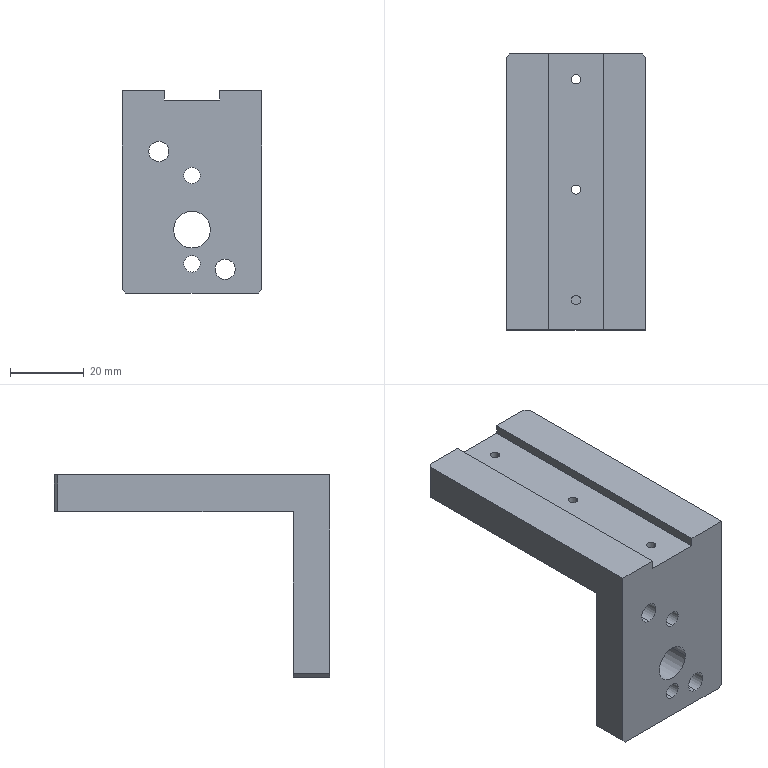Component | SolidWorks | CCDJSGrippingCylinderAngleAluminum01-1 | 1 solid | 33 faces | box 38 x 75 x 55 mm | volume 41060 mm3 | plane 17 | cylinder 16 | commonest cylinder face diameters 2.5 x6 4.5 x4 5.5 x4 10 x2
STEP:
#1=COLOUR_RGB('',0.7922,0.8196,0.9333);
#2=FILL_AREA_STYLE_COLOUR('',#1);
#3=FILL_AREA_STYLE('',(#2));
#4=SURFACE_STYLE_FILL_AREA(#3);
#5=SURFACE_SIDE_STYLE('',(#4));
#6=SURFACE_STYLE_USAGE(.BOTH.,#5);
#7=PRESENTATION_STYLE_ASSIGNMENT((#6));
#8=CARTESIAN_POINT('',(-6.256,14.188,-4.54));
#9=VERTEX_POINT('',#8);
#10=CARTESIAN_POINT('',(-6.256,14.188,-4.363));
#11=VERTEX_POINT('',#10);
#12=CARTESIAN_POINT('',(-6.256,14.188,-4.452));
#13=DIRECTION('',(-0.,1.,0.));
#14=DIRECTION('',(0.,0.,1.));
#15=AXIS2_PLACEMENT_3D('',#12,#13,#14);
#16=CIRCLE('',#15,0.08858);
#17=EDGE_CURVE('',#9,#11,#16,.T.);
#18=ORIENTED_EDGE('',*,*,#17,.F.);
#19=CARTESIAN_POINT('',(-6.256,14.581,-4.54));
#20=VERTEX_POINT('',#19);
#21=CARTESIAN_POINT('',(-6.256,14.188,-4.54));
#22=DIRECTION('',(-0.,1.,0.));
#23=VECTOR('',#22,39.37);
#24=LINE('',#21,#23);
#25=EDGE_CURVE('',#9,#20,#24,.T.);
#26=ORIENTED_EDGE('',*,*,#25,.T.);
#27=CARTESIAN_POINT('',(-6.256,14.581,-4.363));
#28=VERTEX_POINT('',#27);
#29=CARTESIAN_POINT('',(-6.256,14.581,-4.452));
#30=DIRECTION('',(-0.,1.,0.));
#31=DIRECTION('',(0.,0.,1.));
#32=AXIS2_PLACEMENT_3D('',#29,#30,#31);
#33=CIRCLE('',#32,0.08858);
#34=EDGE_CURVE('',#20,#28,#33,.T.);
#35=ORIENTED_EDGE('',*,*,#34,.T.);
#36=CARTESIAN_POINT('',(-6.256,14.188,-4.363));
#37=DIRECTION('',(-0.,1.,0.));
#38=VECTOR('',#37,39.37);
#39=LINE('',#36,#38);
#40=EDGE_CURVE('',#11,#28,#39,.T.);
#41=ORIENTED_EDGE('',*,*,#40,.F.);
#42=EDGE_LOOP('',(#18,#26,#35,#41));
#43=FACE_OUTER_BOUND('',#42,.T.);
#44=CARTESIAN_POINT('',(-6.256,14.188,-4.452));
#45=DIRECTION('',(-0.,1.,0.));
#46=DIRECTION('',(0.,0.,1.));
#47=AXIS2_PLACEMENT_3D('',#44,#45,#46);
#48=CYLINDRICAL_SURFACE('',#47,0.08858);
#49=ADVANCED_FACE('',(#43),#48,.F.);
#50=CARTESIAN_POINT('',(-6.256,14.188,-5.485));
#51=VERTEX_POINT('',#50);
#52=CARTESIAN_POINT('',(-6.256,14.188,-5.308));
#53=VERTEX_POINT('',#52);
#54=CARTESIAN_POINT('',(-6.256,14.188,-5.396));
#55=DIRECTION('',(-0.,1.,0.));
#56=DIRECTION('',(0.,0.,1.));
#57=AXIS2_PLACEMENT_3D('',#54,#55,#56);
#58=CIRCLE('',#57,0.08858);
#59=EDGE_CURVE('',#51,#53,#58,.T.);
#60=ORIENTED_EDGE('',*,*,#59,.F.);
#61=CARTESIAN_POINT('',(-6.256,14.581,-5.485));
#62=VERTEX_POINT('',#61);
#63=CARTESIAN_POINT('',(-6.256,14.188,-5.485));
#64=DIRECTION('',(-0.,1.,0.));
#65=VECTOR('',#64,39.37);
#66=LINE('',#63,#65);
#67=EDGE_CURVE('',#51,#62,#66,.T.);
#68=ORIENTED_EDGE('',*,*,#67,.T.);
#69=CARTESIAN_POINT('',(-6.256,14.581,-5.308));
#70=VERTEX_POINT('',#69);
#71=CARTESIAN_POINT('',(-6.256,14.581,-5.396));
#72=DIRECTION('',(-0.,1.,0.));
#73=DIRECTION('',(0.,0.,1.));
#74=AXIS2_PLACEMENT_3D('',#71,#72,#73);
#75=CIRCLE('',#74,0.08858);
#76=EDGE_CURVE('',#62,#70,#75,.T.);
#77=ORIENTED_EDGE('',*,*,#76,.T.);
#78=CARTESIAN_POINT('',(-6.256,14.188,-5.308));
#79=DIRECTION('',(-0.,1.,0.));
#80=VECTOR('',#79,39.37);
#81=LINE('',#78,#80);
#82=EDGE_CURVE('',#53,#70,#81,.T.);
#83=ORIENTED_EDGE('',*,*,#82,.F.);
#84=EDGE_LOOP('',(#60,#68,#77,#83));
#85=FACE_OUTER_BOUND('',#84,.T.);
#86=CARTESIAN_POINT('',(-6.256,14.188,-5.396));
#87=DIRECTION('',(-0.,1.,0.));
#88=DIRECTION('',(0.,0.,1.));
#89=AXIS2_PLACEMENT_3D('',#86,#87,#88);
#90=CYLINDRICAL_SURFACE('',#89,0.08858);
#91=ADVANCED_FACE('',(#85),#90,.F.);
#92=CARTESIAN_POINT('',(-5.902,14.188,-5.564));
#93=VERTEX_POINT('',#92);
#94=CARTESIAN_POINT('',(-5.902,14.188,-5.347));
#95=VERTEX_POINT('',#94);
#96=CARTESIAN_POINT('',(-5.902,14.188,-5.456));
#97=DIRECTION('',(-0.,1.,0.));
#98=DIRECTION('',(1.,0.,0.));
#99=AXIS2_PLACEMENT_3D('',#96,#97,#98);
#100=CIRCLE('',#99,0.1083);
#101=EDGE_CURVE('',#93,#95,#100,.T.);
#102=ORIENTED_EDGE('',*,*,#101,.F.);
#103=CARTESIAN_POINT('',(-5.902,14.581,-5.564));
#104=VERTEX_POINT('',#103);
#105=CARTESIAN_POINT('',(-5.902,13.755,-5.564));
#106=DIRECTION('',(-0.,1.,0.));
#107=VECTOR('',#106,39.37);
#108=LINE('',#105,#107);
#109=EDGE_CURVE('',#93,#104,#108,.T.);
#110=ORIENTED_EDGE('',*,*,#109,.T.);
#111=CARTESIAN_POINT('',(-5.902,14.581,-5.347));
#112=VERTEX_POINT('',#111);
#113=CARTESIAN_POINT('',(-5.902,14.581,-5.456));
#114=DIRECTION('',(-0.,1.,0.));
#115=DIRECTION('',(0.,0.,1.));
#116=AXIS2_PLACEMENT_3D('',#113,#114,#115);
#117=CIRCLE('',#116,0.1083);
#118=EDGE_CURVE('',#104,#112,#117,.T.);
#119=ORIENTED_EDGE('',*,*,#118,.T.);
#120=CARTESIAN_POINT('',(-5.902,13.755,-5.347));
#121=DIRECTION('',(-0.,1.,0.));
#122=VECTOR('',#121,39.37);
#123=LINE('',#120,#122);
#124=EDGE_CURVE('',#95,#112,#123,.T.);
#125=ORIENTED_EDGE('',*,*,#124,.F.);
#126=EDGE_LOOP('',(#102,#110,#119,#125));
#127=FACE_OUTER_BOUND('',#126,.T.);
#128=CARTESIAN_POINT('',(-5.902,13.755,-5.456));
#129=DIRECTION('',(-0.,1.,0.));
#130=DIRECTION('',(0.,0.,1.));
#131=AXIS2_PLACEMENT_3D('',#128,#129,#130);
#132=CYLINDRICAL_SURFACE('',#131,0.1083);
#133=ADVANCED_FACE('',(#127),#132,.F.);
#134=CARTESIAN_POINT('',(-6.61,14.188,-4.304));
#135=VERTEX_POINT('',#134);
#136=CARTESIAN_POINT('',(-6.61,14.188,-4.087));
#137=VERTEX_POINT('',#136);
#138=CARTESIAN_POINT('',(-6.61,14.188,-4.196));
#139=DIRECTION('',(-0.,1.,0.));
#140=DIRECTION('',(1.,0.,0.));
#141=AXIS2_PLACEMENT_3D('',#138,#139,#140);
#142=CIRCLE('',#141,0.1083);
#143=EDGE_CURVE('',#135,#137,#142,.T.);
#144=ORIENTED_EDGE('',*,*,#143,.F.);
#145=CARTESIAN_POINT('',(-6.61,14.581,-4.304));
#146=VERTEX_POINT('',#145);
#147=CARTESIAN_POINT('',(-6.61,13.755,-4.304));
#148=DIRECTION('',(-0.,1.,0.));
#149=VECTOR('',#148,39.37);
#150=LINE('',#147,#149);
#151=EDGE_CURVE('',#135,#146,#150,.T.);
#152=ORIENTED_EDGE('',*,*,#151,.T.);
#153=CARTESIAN_POINT('',(-6.61,14.581,-4.087));
#154=VERTEX_POINT('',#153);
#155=CARTESIAN_POINT('',(-6.61,14.581,-4.196));
#156=DIRECTION('',(-0.,1.,0.));
#157=DIRECTION('',(0.,0.,1.));
#158=AXIS2_PLACEMENT_3D('',#155,#156,#157);
#159=CIRCLE('',#158,0.1083);
#160=EDGE_CURVE('',#146,#154,#159,.T.);
#161=ORIENTED_EDGE('',*,*,#160,.T.);
#162=CARTESIAN_POINT('',(-6.61,13.755,-4.087));
#163=DIRECTION('',(-0.,1.,0.));
#164=VECTOR('',#163,39.37);
#165=LINE('',#162,#164);
#166=EDGE_CURVE('',#137,#154,#165,.T.);
#167=ORIENTED_EDGE('',*,*,#166,.F.);
#168=EDGE_LOOP('',(#144,#152,#161,#167));
#169=FACE_OUTER_BOUND('',#168,.T.);
#170=CARTESIAN_POINT('',(-6.61,13.755,-4.196));
#171=DIRECTION('',(-0.,1.,0.));
#172=DIRECTION('',(0.,0.,1.));
#173=AXIS2_PLACEMENT_3D('',#170,#171,#172);
#174=CYLINDRICAL_SURFACE('',#173,0.1083);
#175=ADVANCED_FACE('',(#169),#174,.F.);
#176=CARTESIAN_POINT('',(-6.207,14.506,-3.644));
#177=VERTEX_POINT('',#176);
#178=CARTESIAN_POINT('',(-6.305,14.506,-3.644));
#179=VERTEX_POINT('',#178);
#180=CARTESIAN_POINT('',(-6.256,14.506,-3.644));
#181=DIRECTION('',(0.,0.,-1.));
#182=DIRECTION('',(-1.,0.,0.));
#183=AXIS2_PLACEMENT_3D('',#180,#181,#182);
#184=CIRCLE('',#183,0.04921);
#185=EDGE_CURVE('',#177,#179,#184,.T.);
#186=ORIENTED_EDGE('',*,*,#185,.F.);
#187=CARTESIAN_POINT('',(-6.207,14.506,-3.94));
#188=VERTEX_POINT('',#187);
#189=CARTESIAN_POINT('',(-6.207,14.506,-3.94));
#190=DIRECTION('',(0.,0.,-1.));
#191=VECTOR('',#190,39.37);
#192=LINE('',#189,#191);
#193=EDGE_CURVE('',#177,#188,#192,.T.);
#194=ORIENTED_EDGE('',*,*,#193,.T.);
#195=CARTESIAN_POINT('',(-6.305,14.506,-3.94));
#196=VERTEX_POINT('',#195);
#197=CARTESIAN_POINT('',(-6.256,14.506,-3.94));
#198=DIRECTION('',(0.,0.,-1.));
#199=DIRECTION('',(-1.,0.,0.));
#200=AXIS2_PLACEMENT_3D('',#197,#198,#199);
#201=CIRCLE('',#200,0.04921);
#202=EDGE_CURVE('',#188,#196,#201,.T.);
#203=ORIENTED_EDGE('',*,*,#202,.T.);
#204=CARTESIAN_POINT('',(-6.305,14.506,-3.94));
#205=DIRECTION('',(0.,0.,-1.));
#206=VECTOR('',#205,39.37);
#207=LINE('',#204,#206);
#208=EDGE_CURVE('',#179,#196,#207,.T.);
#209=ORIENTED_EDGE('',*,*,#208,.F.);
#210=EDGE_LOOP('',(#186,#194,#203,#209));
#211=FACE_OUTER_BOUND('',#210,.T.);
#212=CARTESIAN_POINT('',(-6.256,14.506,-3.94));
#213=DIRECTION('',(0.,0.,-1.));
#214=DIRECTION('',(-1.,0.,0.));
#215=AXIS2_PLACEMENT_3D('',#212,#213,#214);
#216=CYLINDRICAL_SURFACE('',#215,0.04921);
#217=ADVANCED_FACE('',(#211),#216,.F.);
#218=CARTESIAN_POINT('',(-6.207,15.688,-3.644));
#219=VERTEX_POINT('',#218);
#220=CARTESIAN_POINT('',(-6.305,15.688,-3.644));
#221=VERTEX_POINT('',#220);
#222=CARTESIAN_POINT('',(-6.256,15.688,-3.644));
#223=DIRECTION('',(0.,0.,-1.));
#224=DIRECTION('',(-1.,0.,0.));
#225=AXIS2_PLACEMENT_3D('',#222,#223,#224);
#226=CIRCLE('',#225,0.04921);
#227=EDGE_CURVE('',#219,#221,#226,.T.);
#228=ORIENTED_EDGE('',*,*,#227,.F.);
#229=CARTESIAN_POINT('',(-6.207,15.688,-3.94));
#230=VERTEX_POINT('',#229);
#231=CARTESIAN_POINT('',(-6.207,15.688,-3.94));
#232=DIRECTION('',(0.,0.,-1.));
#233=VECTOR('',#232,39.37);
#234=LINE('',#231,#233);
#235=EDGE_CURVE('',#219,#230,#234,.T.);
#236=ORIENTED_EDGE('',*,*,#235,.T.);
#237=CARTESIAN_POINT('',(-6.305,15.688,-3.94));
#238=VERTEX_POINT('',#237);
#239=CARTESIAN_POINT('',(-6.256,15.688,-3.94));
#240=DIRECTION('',(0.,0.,-1.));
#241=DIRECTION('',(-1.,0.,0.));
#242=AXIS2_PLACEMENT_3D('',#239,#240,#241);
#243=CIRCLE('',#242,0.04921);
#244=EDGE_CURVE('',#230,#238,#243,.T.);
#245=ORIENTED_EDGE('',*,*,#244,.T.);
#246=CARTESIAN_POINT('',(-6.305,15.688,-3.94));
#247=DIRECTION('',(0.,0.,-1.));
#248=VECTOR('',#247,39.37);
#249=LINE('',#246,#248);
#250=EDGE_CURVE('',#221,#238,#249,.T.);
#251=ORIENTED_EDGE('',*,*,#250,.F.);
#252=EDGE_LOOP('',(#228,#236,#245,#251));
#253=FACE_OUTER_BOUND('',#252,.T.);
#254=CARTESIAN_POINT('',(-6.256,15.688,-3.94));
#255=DIRECTION('',(0.,0.,-1.));
#256=DIRECTION('',(-1.,0.,0.));
#257=AXIS2_PLACEMENT_3D('',#254,#255,#256);
#258=CYLINDRICAL_SURFACE('',#257,0.04921);
#259=ADVANCED_FACE('',(#253),#258,.F.);
#260=CARTESIAN_POINT('',(-6.207,16.869,-3.644));
#261=VERTEX_POINT('',#260);
#262=CARTESIAN_POINT('',(-6.305,16.869,-3.644));
#263=VERTEX_POINT('',#262);
#264=CARTESIAN_POINT('',(-6.256,16.869,-3.644));
#265=DIRECTION('',(0.,0.,-1.));
#266=DIRECTION('',(-1.,0.,0.));
#267=AXIS2_PLACEMENT_3D('',#264,#265,#266);
#268=CIRCLE('',#267,0.04921);
#269=EDGE_CURVE('',#261,#263,#268,.T.);
#270=ORIENTED_EDGE('',*,*,#269,.F.);
#271=CARTESIAN_POINT('',(-6.207,16.869,-3.94));
#272=VERTEX_POINT('',#271);
#273=CARTESIAN_POINT('',(-6.207,16.869,-3.94));
#274=DIRECTION('',(0.,0.,-1.));
#275=VECTOR('',#274,39.37);
#276=LINE('',#273,#275);
#277=EDGE_CURVE('',#261,#272,#276,.T.);
#278=ORIENTED_EDGE('',*,*,#277,.T.);
#279=CARTESIAN_POINT('',(-6.305,16.869,-3.94));
#280=VERTEX_POINT('',#279);
#281=CARTESIAN_POINT('',(-6.256,16.869,-3.94));
#282=DIRECTION('',(0.,0.,-1.));
#283=DIRECTION('',(-1.,0.,0.));
#284=AXIS2_PLACEMENT_3D('',#281,#282,#283);
#285=CIRCLE('',#284,0.04921);
#286=EDGE_CURVE('',#272,#280,#285,.T.);
#287=ORIENTED_EDGE('',*,*,#286,.T.);
#288=CARTESIAN_POINT('',(-6.305,16.869,-3.94));
#289=DIRECTION('',(0.,0.,-1.));
#290=VECTOR('',#289,39.37);
#291=LINE('',#288,#290);
#292=EDGE_CURVE('',#263,#280,#291,.T.);
#293=ORIENTED_EDGE('',*,*,#292,.F.);
#294=EDGE_LOOP('',(#270,#278,#287,#293));
#295=FACE_OUTER_BOUND('',#294,.T.);
#296=CARTESIAN_POINT('',(-6.256,16.869,-3.94));
#297=DIRECTION('',(0.,0.,-1.));
#298=DIRECTION('',(-1.,0.,0.));
#299=AXIS2_PLACEMENT_3D('',#296,#297,#298);
#300=CYLINDRICAL_SURFACE('',#299,0.04921);
#301=ADVANCED_FACE('',(#295),#300,.F.);
#302=CARTESIAN_POINT('',(-6.453,14.188,-5.032));
#303=VERTEX_POINT('',#302);
#304=CARTESIAN_POINT('',(-6.059,14.188,-5.032));
#305=VERTEX_POINT('',#304);
#306=CARTESIAN_POINT('',(-6.256,14.188,-5.032));
#307=DIRECTION('',(-0.,1.,0.));
#308=DIRECTION('',(1.,0.,0.));
#309=AXIS2_PLACEMENT_3D('',#306,#307,#308);
#310=CIRCLE('',#309,0.1969);
#311=EDGE_CURVE('',#303,#305,#310,.T.);
#312=ORIENTED_EDGE('',*,*,#311,.F.);
#313=CARTESIAN_POINT('',(-6.453,14.581,-5.032));
#314=VERTEX_POINT('',#313);
#315=CARTESIAN_POINT('',(-6.453,14.581,-5.032));
#316=DIRECTION('',(-0.,1.,0.));
#317=VECTOR('',#316,39.37);
#318=LINE('',#315,#317);
#319=EDGE_CURVE('',#303,#314,#318,.T.);
#320=ORIENTED_EDGE('',*,*,#319,.T.);
#321=CARTESIAN_POINT('',(-6.059,14.581,-5.032));
#322=VERTEX_POINT('',#321);
#323=CARTESIAN_POINT('',(-6.256,14.581,-5.032));
#324=DIRECTION('',(-0.,1.,0.));
#325=DIRECTION('',(1.,0.,0.));
#326=AXIS2_PLACEMENT_3D('',#323,#324,#325);
#327=CIRCLE('',#326,0.1969);
#328=EDGE_CURVE('',#314,#322,#327,.T.);
#329=ORIENTED_EDGE('',*,*,#328,.T.);
#330=CARTESIAN_POINT('',(-6.059,14.581,-5.032));
#331=DIRECTION('',(-0.,1.,0.));
#332=VECTOR('',#331,39.37);
#333=LINE('',#330,#332);
#334=EDGE_CURVE('',#305,#322,#333,.T.);
#335=ORIENTED_EDGE('',*,*,#334,.F.);
#336=EDGE_LOOP('',(#312,#320,#329,#335));
#337=FACE_OUTER_BOUND('',#336,.T.);
#338=CARTESIAN_POINT('',(-6.256,14.581,-5.032));
#339=DIRECTION('',(-0.,1.,0.));
#340=DIRECTION('',(1.,0.,0.));
#341=AXIS2_PLACEMENT_3D('',#338,#339,#340);
#342=CYLINDRICAL_SURFACE('',#341,0.1969);
#343=ADVANCED_FACE('',(#337),#342,.F.);
#344=CARTESIAN_POINT('',(-5.508,17.101,-3.546));
#345=VERTEX_POINT('',#344);
#346=CARTESIAN_POINT('',(-5.508,14.188,-3.546));
#347=VERTEX_POINT('',#346);
#348=CARTESIAN_POINT('',(-5.508,17.14,-3.546));
#349=DIRECTION('',(0.,-1.,-0.));
#350=VECTOR('',#349,39.37);
#351=LINE('',#348,#350);
#352=EDGE_CURVE('',#345,#347,#351,.T.);
#353=ORIENTED_EDGE('',*,*,#352,.F.);
#354=CARTESIAN_POINT('',(-5.547,17.14,-3.546));
#355=VERTEX_POINT('',#354);
#356=CARTESIAN_POINT('',(-5.508,17.101,-3.546));
#357=DIRECTION('',(-0.7071,0.7071,0.));
#358=VECTOR('',#357,39.37);
#359=LINE('',#356,#358);
#360=EDGE_CURVE('',#345,#355,#359,.T.);
#361=ORIENTED_EDGE('',*,*,#360,.T.);
#362=CARTESIAN_POINT('',(-5.959,17.14,-3.546));
#363=VERTEX_POINT('',#362);
#364=CARTESIAN_POINT('',(-5.508,17.14,-3.546));
#365=DIRECTION('',(-1.,-0.,0.));
#366=VECTOR('',#365,39.37);
#367=LINE('',#364,#366);
#368=EDGE_CURVE('',#355,#363,#367,.T.);
#369=ORIENTED_EDGE('',*,*,#368,.T.);
#370=CARTESIAN_POINT('',(-5.959,14.188,-3.546));
#371=VERTEX_POINT('',#370);
#372=CARTESIAN_POINT('',(-5.959,17.14,-3.546));
#373=DIRECTION('',(0.,-1.,-0.));
#374=VECTOR('',#373,39.37);
#375=LINE('',#372,#374);
#376=EDGE_CURVE('',#363,#371,#375,.T.);
#377=ORIENTED_EDGE('',*,*,#376,.T.);
#378=CARTESIAN_POINT('',(-5.508,14.188,-3.546));
#379=DIRECTION('',(-1.,-0.,0.));
#380=VECTOR('',#379,39.37);
#381=LINE('',#378,#380);
#382=EDGE_CURVE('',#347,#371,#381,.T.);
#383=ORIENTED_EDGE('',*,*,#382,.F.);
#384=EDGE_LOOP('',(#353,#361,#369,#377,#383));
#385=FACE_OUTER_BOUND('',#384,.T.);
#386=CARTESIAN_POINT('',(-5.508,17.14,-3.546));
#387=DIRECTION('',(-0.,0.,-1.));
#388=DIRECTION('',(-0.,1.,0.));
#389=AXIS2_PLACEMENT_3D('',#386,#387,#388);
#390=PLANE('',#389);
#391=ADVANCED_FACE('',(#385),#390,.F.);
#392=CARTESIAN_POINT('',(-6.256,14.581,-4.452));
#393=DIRECTION('',(-0.,1.,0.));
#394=DIRECTION('',(0.,0.,1.));
#395=AXIS2_PLACEMENT_3D('',#392,#393,#394);
#396=CIRCLE('',#395,0.08858);
#397=EDGE_CURVE('',#28,#20,#396,.T.);
#398=ORIENTED_EDGE('',*,*,#397,.F.);
#399=ORIENTED_EDGE('',*,*,#34,.F.);
#400=EDGE_LOOP('',(#398,#399));
#401=FACE_BOUND('',#400,.T.);
#402=CARTESIAN_POINT('',(-6.256,14.581,-5.396));
#403=DIRECTION('',(-0.,1.,0.));
#404=DIRECTION('',(0.,0.,1.));
#405=AXIS2_PLACEMENT_3D('',#402,#403,#404);
#406=CIRCLE('',#405,0.08858);
#407=EDGE_CURVE('',#70,#62,#406,.T.);
#408=ORIENTED_EDGE('',*,*,#407,.F.);
#409=ORIENTED_EDGE('',*,*,#76,.F.);
#410=EDGE_LOOP('',(#408,#409));
#411=FACE_BOUND('',#410,.T.);
#412=CARTESIAN_POINT('',(-5.902,14.581,-5.456));
#413=DIRECTION('',(-0.,1.,0.));
#414=DIRECTION('',(0.,0.,1.));
#415=AXIS2_PLACEMENT_3D('',#412,#413,#414);
#416=CIRCLE('',#415,0.1083);
#417=EDGE_CURVE('',#112,#104,#416,.T.);
#418=ORIENTED_EDGE('',*,*,#417,.F.);
#419=ORIENTED_EDGE('',*,*,#118,.F.);
#420=EDGE_LOOP('',(#418,#419));
#421=FACE_BOUND('',#420,.T.);
#422=CARTESIAN_POINT('',(-6.61,14.581,-4.196));
#423=DIRECTION('',(-0.,1.,0.));
#424=DIRECTION('',(0.,0.,1.));
#425=AXIS2_PLACEMENT_3D('',#422,#423,#424);
#426=CIRCLE('',#425,0.1083);
#427=EDGE_CURVE('',#154,#146,#426,.T.);
#428=ORIENTED_EDGE('',*,*,#427,.F.);
#429=ORIENTED_EDGE('',*,*,#160,.F.);
#430=EDGE_LOOP('',(#428,#429));
#431=FACE_BOUND('',#430,.T.);
#432=CARTESIAN_POINT('',(-6.256,14.581,-5.032));
#433=DIRECTION('',(-0.,1.,0.));
#434=DIRECTION('',(1.,0.,0.));
#435=AXIS2_PLACEMENT_3D('',#432,#433,#434);
#436=CIRCLE('',#435,0.1969);
#437=EDGE_CURVE('',#322,#314,#436,.T.);
#438=ORIENTED_EDGE('',*,*,#437,.F.);
#439=ORIENTED_EDGE('',*,*,#328,.F.);
#440=EDGE_LOOP('',(#438,#439));
#441=FACE_BOUND('',#440,.T.);
#442=CARTESIAN_POINT('',(-5.508,14.581,-5.672));
#443=VERTEX_POINT('',#442);
#444=CARTESIAN_POINT('',(-5.508,14.581,-3.94));
#445=VERTEX_POINT('',#444);
#446=CARTESIAN_POINT('',(-5.508,14.581,-5.711));
#447=DIRECTION('',(0.,-0.,1.));
#448=VECTOR('',#447,39.37);
#449=LINE('',#446,#448);
#450=EDGE_CURVE('',#443,#445,#449,.T.);
#451=ORIENTED_EDGE('',*,*,#450,.F.);
#452=CARTESIAN_POINT('',(-5.547,14.581,-5.711));
#453=VERTEX_POINT('',#452);
#454=CARTESIAN_POINT('',(-5.508,14.581,-5.672));
#455=DIRECTION('',(-0.7071,-0.,-0.7071));
#456=VECTOR('',#455,39.37);
#457=LINE('',#454,#456);
#458=EDGE_CURVE('',#443,#453,#457,.T.);
#459=ORIENTED_EDGE('',*,*,#458,.T.);
#460=CARTESIAN_POINT('',(-6.965,14.581,-5.711));
#461=VERTEX_POINT('',#460);
#462=CARTESIAN_POINT('',(-5.508,14.581,-5.711));
#463=DIRECTION('',(-1.,-0.,0.));
#464=VECTOR('',#463,39.37);
#465=LINE('',#462,#464);
#466=EDGE_CURVE('',#453,#461,#465,.T.);
#467=ORIENTED_EDGE('',*,*,#466,.T.);
#468=CARTESIAN_POINT('',(-7.004,14.581,-5.672));
#469=VERTEX_POINT('',#468);
#470=CARTESIAN_POINT('',(-6.965,14.581,-5.711));
#471=DIRECTION('',(-0.7071,-0.,0.7071));
#472=VECTOR('',#471,39.37);
#473=LINE('',#470,#472);
#474=EDGE_CURVE('',#461,#469,#473,.T.);
#475=ORIENTED_EDGE('',*,*,#474,.T.);
#476=CARTESIAN_POINT('',(-7.004,14.581,-3.94));
#477=VERTEX_POINT('',#476);
#478=CARTESIAN_POINT('',(-7.004,14.581,-5.711));
#479=DIRECTION('',(0.,-0.,1.));
#480=VECTOR('',#479,39.37);
#481=LINE('',#478,#480);
#482=EDGE_CURVE('',#469,#477,#481,.T.);
#483=ORIENTED_EDGE('',*,*,#482,.T.);
#484=CARTESIAN_POINT('',(-5.508,14.581,-3.94));
#485=DIRECTION('',(-1.,-0.,0.));
#486=VECTOR('',#485,39.37);
#487=LINE('',#484,#486);
#488=EDGE_CURVE('',#445,#477,#487,.T.);
#489=ORIENTED_EDGE('',*,*,#488,.F.);
#490=EDGE_LOOP('',(#451,#459,#467,#475,#483,#489));
#491=FACE_OUTER_BOUND('',#490,.T.);
#492=CARTESIAN_POINT('',(-5.508,14.581,-5.711));
#493=DIRECTION('',(0.,-1.,-0.));
#494=DIRECTION('',(-0.,0.,-1.));
#495=AXIS2_PLACEMENT_3D('',#492,#493,#494);
#496=PLANE('',#495);
#497=ADVANCED_FACE('',(#401,#411,#421,#431,#441,#491),#496,.F.);
#498=CARTESIAN_POINT('',(-6.256,15.688,-3.94));
#499=DIRECTION('',(0.,0.,-1.));
#500=DIRECTION('',(-1.,0.,0.));
#501=AXIS2_PLACEMENT_3D('',#498,#499,#500);
#502=CIRCLE('',#501,0.04921);
#503=EDGE_CURVE('',#238,#230,#502,.T.);
#504=ORIENTED_EDGE('',*,*,#503,.F.);
#505=ORIENTED_EDGE('',*,*,#244,.F.);
#506=EDGE_LOOP('',(#504,#505));
#507=FACE_BOUND('',#506,.T.);
#508=CARTESIAN_POINT('',(-6.256,16.869,-3.94));
#509=DIRECTION('',(0.,0.,-1.));
#510=DIRECTION('',(-1.,0.,0.));
#511=AXIS2_PLACEMENT_3D('',#508,#509,#510);
#512=CIRCLE('',#511,0.04921);
#513=EDGE_CURVE('',#280,#272,#512,.T.);
#514=ORIENTED_EDGE('',*,*,#513,.F.);
#515=ORIENTED_EDGE('',*,*,#286,.F.);
#516=EDGE_LOOP('',(#514,#515));
#517=FACE_BOUND('',#516,.T.);
#518=CARTESIAN_POINT('',(-7.004,17.101,-3.94));
#519=VERTEX_POINT('',#518);
#520=CARTESIAN_POINT('',(-7.004,14.581,-3.94));
#521=DIRECTION('',(-0.,1.,0.));
#522=VECTOR('',#521,39.37);
#523=LINE('',#520,#522);
#524=EDGE_CURVE('',#477,#519,#523,.T.);
#525=ORIENTED_EDGE('',*,*,#524,.T.);
#526=CARTESIAN_POINT('',(-6.965,17.14,-3.94));
#527=VERTEX_POINT('',#526);
#528=CARTESIAN_POINT('',(-6.965,17.14,-3.94));
#529=DIRECTION('',(0.7071,0.7071,0.));
#530=VECTOR('',#529,39.37);
#531=LINE('',#528,#530);
#532=EDGE_CURVE('',#519,#527,#531,.T.);
#533=ORIENTED_EDGE('',*,*,#532,.T.);
#534=CARTESIAN_POINT('',(-5.547,17.14,-3.94));
#535=VERTEX_POINT('',#534);
#536=CARTESIAN_POINT('',(-5.508,17.14,-3.94));
#537=DIRECTION('',(-1.,-0.,0.));
#538=VECTOR('',#537,39.37);
#539=LINE('',#536,#538);
#540=EDGE_CURVE('',#535,#527,#539,.T.);
#541=ORIENTED_EDGE('',*,*,#540,.F.);
#542=CARTESIAN_POINT('',(-5.508,17.101,-3.94));
#543=VERTEX_POINT('',#542);
#544=CARTESIAN_POINT('',(-5.508,17.101,-3.94));
#545=DIRECTION('',(0.7071,-0.7071,0.));
#546=VECTOR('',#545,39.37);
#547=LINE('',#544,#546);
#548=EDGE_CURVE('',#535,#543,#547,.T.);
#549=ORIENTED_EDGE('',*,*,#548,.T.);
#550=CARTESIAN_POINT('',(-5.508,14.581,-3.94));
#551=DIRECTION('',(-0.,1.,0.));
#552=VECTOR('',#551,39.37);
#553=LINE('',#550,#552);
#554=EDGE_CURVE('',#445,#543,#553,.T.);
#555=ORIENTED_EDGE('',*,*,#554,.F.);
#556=ORIENTED_EDGE('',*,*,#488,.T.);
#557=EDGE_LOOP('',(#525,#533,#541,#549,#555,#556));
#558=FACE_OUTER_BOUND('',#557,.T.);
#559=CARTESIAN_POINT('',(-5.508,14.581,-3.94));
#560=DIRECTION('',(0.,0.,1.));
#561=DIRECTION('',(1.,0.,0.));
#562=AXIS2_PLACEMENT_3D('',#559,#560,#561);
#563=PLANE('',#562);
#564=ADVANCED_FACE('',(#507,#517,#558),#563,.F.);
#565=ORIENTED_EDGE('',*,*,#540,.T.);
#566=CARTESIAN_POINT('',(-6.965,17.14,-3.546));
#567=VERTEX_POINT('',#566);
#568=CARTESIAN_POINT('',(-6.965,17.14,-3.546));
#569=DIRECTION('',(0.,0.,1.));
#570=VECTOR('',#569,39.37);
#571=LINE('',#568,#570);
#572=EDGE_CURVE('',#527,#567,#571,.T.);
#573=ORIENTED_EDGE('',*,*,#572,.T.);
#574=CARTESIAN_POINT('',(-6.553,17.14,-3.546));
#575=VERTEX_POINT('',#574);
#576=CARTESIAN_POINT('',(-5.508,17.14,-3.546));
#577=DIRECTION('',(-1.,-0.,0.));
#578=VECTOR('',#577,39.37);
#579=LINE('',#576,#578);
#580=EDGE_CURVE('',#575,#567,#579,.T.);
#581=ORIENTED_EDGE('',*,*,#580,.F.);
#582=CARTESIAN_POINT('',(-6.553,17.14,-3.644));
#583=VERTEX_POINT('',#582);
#584=CARTESIAN_POINT('',(-6.553,17.14,-3.448));
#585=DIRECTION('',(0.,0.,1.));
#586=VECTOR('',#585,39.37);
#587=LINE('',#584,#586);
#588=EDGE_CURVE('',#583,#575,#587,.T.);
#589=ORIENTED_EDGE('',*,*,#588,.F.);
#590=CARTESIAN_POINT('',(-5.959,17.14,-3.644));
#591=VERTEX_POINT('',#590);
#592=CARTESIAN_POINT('',(-5.959,17.14,-3.644));
#593=DIRECTION('',(-1.,-0.,0.));
#594=VECTOR('',#593,39.37);
#595=LINE('',#592,#594);
#596=EDGE_CURVE('',#591,#583,#595,.T.);
#597=ORIENTED_EDGE('',*,*,#596,.F.);
#598=CARTESIAN_POINT('',(-5.959,17.14,-3.448));
#599=DIRECTION('',(0.,0.,-1.));
#600=VECTOR('',#599,39.37);
#601=LINE('',#598,#600);
#602=EDGE_CURVE('',#363,#591,#601,.T.);
#603=ORIENTED_EDGE('',*,*,#602,.F.);
#604=ORIENTED_EDGE('',*,*,#368,.F.);
#605=CARTESIAN_POINT('',(-5.547,17.14,-3.94));
#606=DIRECTION('',(0.,0.,-1.));
#607=VECTOR('',#606,39.37);
#608=LINE('',#605,#607);
#609=EDGE_CURVE('',#355,#535,#608,.T.);
#610=ORIENTED_EDGE('',*,*,#609,.T.);
#611=EDGE_LOOP('',(#565,#573,#581,#589,#597,#603,#604,#610));
#612=FACE_OUTER_BOUND('',#611,.T.);
#613=CARTESIAN_POINT('',(-5.508,17.14,-3.94));
#614=DIRECTION('',(0.,-1.,0.));
#615=DIRECTION('',(-1.,-0.,0.));
#616=AXIS2_PLACEMENT_3D('',#613,#614,#615);
#617=PLANE('',#616);
#618=ADVANCED_FACE('',(#612),#617,.F.);
#619=ORIENTED_EDGE('',*,*,#580,.T.);
#620=CARTESIAN_POINT('',(-7.004,17.101,-3.546));
#621=VERTEX_POINT('',#620);
#622=CARTESIAN_POINT('',(-6.965,17.14,-3.546));
#623=DIRECTION('',(-0.7071,-0.7071,-0.));
#624=VECTOR('',#623,39.37);
#625=LINE('',#622,#624);
#626=EDGE_CURVE('',#567,#621,#625,.T.);
#627=ORIENTED_EDGE('',*,*,#626,.T.);
#628=CARTESIAN_POINT('',(-7.004,14.188,-3.546));
#629=VERTEX_POINT('',#628);
#630=CARTESIAN_POINT('',(-7.004,17.14,-3.546));
#631=DIRECTION('',(0.,-1.,-0.));
#632=VECTOR('',#631,39.37);
#633=LINE('',#630,#632);
#634=EDGE_CURVE('',#621,#629,#633,.T.);
#635=ORIENTED_EDGE('',*,*,#634,.T.);
#636=CARTESIAN_POINT('',(-6.553,14.188,-3.546));
#637=VERTEX_POINT('',#636);
#638=CARTESIAN_POINT('',(-5.508,14.188,-3.546));
#639=DIRECTION('',(-1.,-0.,0.));
#640=VECTOR('',#639,39.37);
#641=LINE('',#638,#640);
#642=EDGE_CURVE('',#637,#629,#641,.T.);
#643=ORIENTED_EDGE('',*,*,#642,.F.);
#644=CARTESIAN_POINT('',(-6.553,17.14,-3.546));
#645=DIRECTION('',(-0.,1.,0.));
#646=VECTOR('',#645,39.37);
#647=LINE('',#644,#646);
#648=EDGE_CURVE('',#637,#575,#647,.T.);
#649=ORIENTED_EDGE('',*,*,#648,.T.);
#650=EDGE_LOOP('',(#619,#627,#635,#643,#649));
#651=FACE_OUTER_BOUND('',#650,.T.);
#652=CARTESIAN_POINT('',(-5.508,17.14,-3.546));
#653=DIRECTION('',(-0.,0.,-1.));
#654=DIRECTION('',(-0.,1.,0.));
#655=AXIS2_PLACEMENT_3D('',#652,#653,#654);
#656=PLANE('',#655);
#657=ADVANCED_FACE('',(#651),#656,.F.);
#658=CARTESIAN_POINT('',(-6.256,14.188,-4.452));
#659=DIRECTION('',(-0.,1.,0.));
#660=DIRECTION('',(0.,0.,1.));
#661=AXIS2_PLACEMENT_3D('',#658,#659,#660);
#662=CIRCLE('',#661,0.08858);
#663=EDGE_CURVE('',#11,#9,#662,.T.);
#664=ORIENTED_EDGE('',*,*,#663,.T.);
#665=ORIENTED_EDGE('',*,*,#17,.T.);
#666=EDGE_LOOP('',(#664,#665));
#667=FACE_BOUND('',#666,.T.);
#668=CARTESIAN_POINT('',(-6.256,14.188,-5.396));
#669=DIRECTION('',(-0.,1.,0.));
#670=DIRECTION('',(0.,0.,1.));
#671=AXIS2_PLACEMENT_3D('',#668,#669,#670);
#672=CIRCLE('',#671,0.08858);
#673=EDGE_CURVE('',#53,#51,#672,.T.);
#674=ORIENTED_EDGE('',*,*,#673,.T.);
#675=ORIENTED_EDGE('',*,*,#59,.T.);
#676=EDGE_LOOP('',(#674,#675));
#677=FACE_BOUND('',#676,.T.);
#678=CARTESIAN_POINT('',(-5.902,14.188,-5.456));
#679=DIRECTION('',(-0.,1.,0.));
#680=DIRECTION('',(1.,0.,0.));
#681=AXIS2_PLACEMENT_3D('',#678,#679,#680);
#682=CIRCLE('',#681,0.1083);
#683=EDGE_CURVE('',#95,#93,#682,.T.);
#684=ORIENTED_EDGE('',*,*,#683,.T.);
#685=ORIENTED_EDGE('',*,*,#101,.T.);
#686=EDGE_LOOP('',(#684,#685));
#687=FACE_BOUND('',#686,.T.);
#688=CARTESIAN_POINT('',(-6.61,14.188,-4.196));
#689=DIRECTION('',(-0.,1.,0.));
#690=DIRECTION('',(1.,0.,0.));
#691=AXIS2_PLACEMENT_3D('',#688,#689,#690);
#692=CIRCLE('',#691,0.1083);
#693=EDGE_CURVE('',#137,#135,#692,.T.);
#694=ORIENTED_EDGE('',*,*,#693,.T.);
#695=ORIENTED_EDGE('',*,*,#143,.T.);
#696=EDGE_LOOP('',(#694,#695));
#697=FACE_BOUND('',#696,.T.);
#698=CARTESIAN_POINT('',(-6.256,14.188,-5.032));
#699=DIRECTION('',(-0.,1.,0.));
#700=DIRECTION('',(1.,0.,0.));
#701=AXIS2_PLACEMENT_3D('',#698,#699,#700);
#702=CIRCLE('',#701,0.1969);
#703=EDGE_CURVE('',#305,#303,#702,.T.);
#704=ORIENTED_EDGE('',*,*,#703,.T.);
#705=ORIENTED_EDGE('',*,*,#311,.T.);
#706=EDGE_LOOP('',(#704,#705));
#707=FACE_BOUND('',#706,.T.);
#708=CARTESIAN_POINT('',(-5.547,14.188,-5.711));
#709=VERTEX_POINT('',#708);
#710=CARTESIAN_POINT('',(-6.965,14.188,-5.711));
#711=VERTEX_POINT('',#710);
#712=CARTESIAN_POINT('',(-5.508,14.188,-5.711));
#713=DIRECTION('',(-1.,-0.,0.));
#714=VECTOR('',#713,39.37);
#715=LINE('',#712,#714);
#716=EDGE_CURVE('',#709,#711,#715,.T.);
#717=ORIENTED_EDGE('',*,*,#716,.F.);
#718=CARTESIAN_POINT('',(-5.508,14.188,-5.672));
#719=VERTEX_POINT('',#718);
#720=CARTESIAN_POINT('',(-5.508,14.188,-5.672));
#721=DIRECTION('',(0.7071,0.,0.7071));
#722=VECTOR('',#721,39.37);
#723=LINE('',#720,#722);
#724=EDGE_CURVE('',#709,#719,#723,.T.);
#725=ORIENTED_EDGE('',*,*,#724,.T.);
#726=CARTESIAN_POINT('',(-5.508,14.188,-3.546));
#727=DIRECTION('',(0.,0.,-1.));
#728=VECTOR('',#727,39.37);
#729=LINE('',#726,#728);
#730=EDGE_CURVE('',#347,#719,#729,.T.);
#731=ORIENTED_EDGE('',*,*,#730,.F.);
#732=ORIENTED_EDGE('',*,*,#382,.T.);
#733=CARTESIAN_POINT('',(-5.959,14.188,-3.644));
#734=VERTEX_POINT('',#733);
#735=CARTESIAN_POINT('',(-5.959,14.188,-3.546));
#736=DIRECTION('',(0.,0.,-1.));
#737=VECTOR('',#736,39.37);
#738=LINE('',#735,#737);
#739=EDGE_CURVE('',#371,#734,#738,.T.);
#740=ORIENTED_EDGE('',*,*,#739,.T.);
#741=CARTESIAN_POINT('',(-6.553,14.188,-3.644));
#742=VERTEX_POINT('',#741);
#743=CARTESIAN_POINT('',(-5.508,14.188,-3.644));
#744=DIRECTION('',(-1.,-0.,0.));
#745=VECTOR('',#744,39.37);
#746=LINE('',#743,#745);
#747=EDGE_CURVE('',#734,#742,#746,.T.);
#748=ORIENTED_EDGE('',*,*,#747,.T.);
#749=CARTESIAN_POINT('',(-6.553,14.188,-3.546));
#750=DIRECTION('',(0.,0.,1.));
#751=VECTOR('',#750,39.37);
#752=LINE('',#749,#751);
#753=EDGE_CURVE('',#742,#637,#752,.T.);
#754=ORIENTED_EDGE('',*,*,#753,.T.);
#755=ORIENTED_EDGE('',*,*,#642,.T.);
#756=CARTESIAN_POINT('',(-7.004,14.188,-5.672));
#757=VERTEX_POINT('',#756);
#758=CARTESIAN_POINT('',(-7.004,14.188,-3.546));
#759=DIRECTION('',(0.,0.,-1.));
#760=VECTOR('',#759,39.37);
#761=LINE('',#758,#760);
#762=EDGE_CURVE('',#629,#757,#761,.T.);
#763=ORIENTED_EDGE('',*,*,#762,.T.);
#764=CARTESIAN_POINT('',(-6.965,14.188,-5.711));
#765=DIRECTION('',(0.7071,0.,-0.7071));
#766=VECTOR('',#765,39.37);
#767=LINE('',#764,#766);
#768=EDGE_CURVE('',#757,#711,#767,.T.);
#769=ORIENTED_EDGE('',*,*,#768,.T.);
#770=EDGE_LOOP('',(#717,#725,#731,#732,#740,#748,#754,#755,#763,#769));
#771=FACE_OUTER_BOUND('',#770,.T.);
#772=CARTESIAN_POINT('',(-5.508,14.188,-3.546));
#773=DIRECTION('',(-0.,1.,0.));
#774=DIRECTION('',(1.,0.,0.));
#775=AXIS2_PLACEMENT_3D('',#772,#773,#774);
#776=PLANE('',#775);
#777=ADVANCED_FACE('',(#667,#677,#687,#697,#707,#771),#776,.F.);
#778=ORIENTED_EDGE('',*,*,#466,.F.);
#779=CARTESIAN_POINT('',(-5.547,14.188,-5.711));
#780=DIRECTION('',(0.,-1.,0.));
#781=VECTOR('',#780,39.37);
#782=LINE('',#779,#781);
#783=EDGE_CURVE('',#453,#709,#782,.T.);
#784=ORIENTED_EDGE('',*,*,#783,.T.);
#785=ORIENTED_EDGE('',*,*,#716,.T.);
#786=CARTESIAN_POINT('',(-6.965,14.581,-5.711));
#787=DIRECTION('',(-0.,1.,0.));
#788=VECTOR('',#787,39.37);
#789=LINE('',#786,#788);
#790=EDGE_CURVE('',#711,#461,#789,.T.);
#791=ORIENTED_EDGE('',*,*,#790,.T.);
#792=EDGE_LOOP('',(#778,#784,#785,#791));
#793=FACE_OUTER_BOUND('',#792,.T.);
#794=CARTESIAN_POINT('',(-5.508,14.188,-5.711));
#795=DIRECTION('',(0.,0.,1.));
#796=DIRECTION('',(1.,0.,0.));
#797=AXIS2_PLACEMENT_3D('',#794,#795,#796);
#798=PLANE('',#797);
#799=ADVANCED_FACE('',(#793),#798,.F.);
#800=ORIENTED_EDGE('',*,*,#730,.T.);
#801=CARTESIAN_POINT('',(-5.508,14.581,-5.672));
#802=DIRECTION('',(-0.,1.,0.));
#803=VECTOR('',#802,39.37);
#804=LINE('',#801,#803);
#805=EDGE_CURVE('',#719,#443,#804,.T.);
#806=ORIENTED_EDGE('',*,*,#805,.T.);
#807=ORIENTED_EDGE('',*,*,#450,.T.);
#808=ORIENTED_EDGE('',*,*,#554,.T.);
#809=CARTESIAN_POINT('',(-5.508,17.101,-3.94));
#810=DIRECTION('',(0.,0.,1.));
#811=VECTOR('',#810,39.37);
#812=LINE('',#809,#811);
#813=EDGE_CURVE('',#543,#345,#812,.T.);
#814=ORIENTED_EDGE('',*,*,#813,.T.);
#815=ORIENTED_EDGE('',*,*,#352,.T.);
#816=EDGE_LOOP('',(#800,#806,#807,#808,#814,#815));
#817=FACE_OUTER_BOUND('',#816,.T.);
#818=CARTESIAN_POINT('',(-5.508,14.581,-3.94));
#819=DIRECTION('',(-1.,-0.,0.));
#820=DIRECTION('',(0.,0.,1.));
#821=AXIS2_PLACEMENT_3D('',#818,#819,#820);
#822=PLANE('',#821);
#823=ADVANCED_FACE('',(#817),#822,.F.);
#824=ORIENTED_EDGE('',*,*,#482,.F.);
#825=CARTESIAN_POINT('',(-7.004,14.188,-5.672));
#826=DIRECTION('',(0.,-1.,0.));
#827=VECTOR('',#826,39.37);
#828=LINE('',#825,#827);
#829=EDGE_CURVE('',#469,#757,#828,.T.);
#830=ORIENTED_EDGE('',*,*,#829,.T.);
#831=ORIENTED_EDGE('',*,*,#762,.F.);
#832=ORIENTED_EDGE('',*,*,#634,.F.);
#833=CARTESIAN_POINT('',(-7.004,17.101,-3.94));
#834=DIRECTION('',(0.,0.,-1.));
#835=VECTOR('',#834,39.37);
#836=LINE('',#833,#835);
#837=EDGE_CURVE('',#621,#519,#836,.T.);
#838=ORIENTED_EDGE('',*,*,#837,.T.);
#839=ORIENTED_EDGE('',*,*,#524,.F.);
#840=EDGE_LOOP('',(#824,#830,#831,#832,#838,#839));
#841=FACE_OUTER_BOUND('',#840,.T.);
#842=CARTESIAN_POINT('',(-7.004,14.581,-3.94));
#843=DIRECTION('',(-1.,-0.,0.));
#844=DIRECTION('',(0.,0.,1.));
#845=AXIS2_PLACEMENT_3D('',#842,#843,#844);
#846=PLANE('',#845);
#847=ADVANCED_FACE('',(#841),#846,.T.);
#848=CARTESIAN_POINT('',(-6.256,14.506,-3.644));
#849=DIRECTION('',(0.,0.,-1.));
#850=DIRECTION('',(-1.,0.,0.));
#851=AXIS2_PLACEMENT_3D('',#848,#849,#850);
#852=CIRCLE('',#851,0.04921);
#853=EDGE_CURVE('',#179,#177,#852,.T.);
#854=ORIENTED_EDGE('',*,*,#853,.T.);
#855=ORIENTED_EDGE('',*,*,#185,.T.);
#856=EDGE_LOOP('',(#854,#855));
#857=FACE_BOUND('',#856,.T.);
#858=CARTESIAN_POINT('',(-6.256,15.688,-3.644));
#859=DIRECTION('',(0.,0.,-1.));
#860=DIRECTION('',(-1.,0.,0.));
#861=AXIS2_PLACEMENT_3D('',#858,#859,#860);
#862=CIRCLE('',#861,0.04921);
#863=EDGE_CURVE('',#221,#219,#862,.T.);
#864=ORIENTED_EDGE('',*,*,#863,.T.);
#865=ORIENTED_EDGE('',*,*,#227,.T.);
#866=EDGE_LOOP('',(#864,#865));
#867=FACE_BOUND('',#866,.T.);
#868=CARTESIAN_POINT('',(-6.256,16.869,-3.644));
#869=DIRECTION('',(0.,0.,-1.));
#870=DIRECTION('',(-1.,0.,0.));
#871=AXIS2_PLACEMENT_3D('',#868,#869,#870);
#872=CIRCLE('',#871,0.04921);
#873=EDGE_CURVE('',#263,#261,#872,.T.);
#874=ORIENTED_EDGE('',*,*,#873,.T.);
#875=ORIENTED_EDGE('',*,*,#269,.T.);
#876=EDGE_LOOP('',(#874,#875));
#877=FACE_BOUND('',#876,.T.);
#878=CARTESIAN_POINT('',(-5.959,12.652,-3.644));
#879=DIRECTION('',(-0.,1.,0.));
#880=VECTOR('',#879,39.37);
#881=LINE('',#878,#880);
#882=EDGE_CURVE('',#734,#591,#881,.T.);
#883=ORIENTED_EDGE('',*,*,#882,.T.);
#884=ORIENTED_EDGE('',*,*,#596,.T.);
#885=CARTESIAN_POINT('',(-6.553,12.652,-3.644));
#886=DIRECTION('',(-0.,1.,0.));
#887=VECTOR('',#886,39.37);
#888=LINE('',#885,#887);
#889=EDGE_CURVE('',#742,#583,#888,.T.);
#890=ORIENTED_EDGE('',*,*,#889,.F.);
#891=ORIENTED_EDGE('',*,*,#747,.F.);
#892=EDGE_LOOP('',(#883,#884,#890,#891));
#893=FACE_OUTER_BOUND('',#892,.T.);
#894=CARTESIAN_POINT('',(-5.959,12.652,-3.644));
#895=DIRECTION('',(0.,0.,-1.));
#896=DIRECTION('',(-1.,-0.,0.));
#897=AXIS2_PLACEMENT_3D('',#894,#895,#896);
#898=PLANE('',#897);
#899=ADVANCED_FACE('',(#857,#867,#877,#893),#898,.F.);
#900=ORIENTED_EDGE('',*,*,#602,.T.);
#901=ORIENTED_EDGE('',*,*,#882,.F.);
#902=ORIENTED_EDGE('',*,*,#739,.F.);
#903=ORIENTED_EDGE('',*,*,#376,.F.);
#904=EDGE_LOOP('',(#900,#901,#902,#903));
#905=FACE_OUTER_BOUND('',#904,.T.);
#906=CARTESIAN_POINT('',(-5.959,12.652,-3.448));
#907=DIRECTION('',(1.,0.,0.));
#908=DIRECTION('',(0.,0.,-1.));
#909=AXIS2_PLACEMENT_3D('',#906,#907,#908);
#910=PLANE('',#909);
#911=ADVANCED_FACE('',(#905),#910,.F.);
#912=ORIENTED_EDGE('',*,*,#753,.F.);
#913=ORIENTED_EDGE('',*,*,#889,.T.);
#914=ORIENTED_EDGE('',*,*,#588,.T.);
#915=ORIENTED_EDGE('',*,*,#648,.F.);
#916=EDGE_LOOP('',(#912,#913,#914,#915));
#917=FACE_OUTER_BOUND('',#916,.T.);
#918=CARTESIAN_POINT('',(-6.553,12.652,-3.448));
#919=DIRECTION('',(-1.,-0.,0.));
#920=DIRECTION('',(0.,0.,1.));
#921=AXIS2_PLACEMENT_3D('',#918,#919,#920);
#922=PLANE('',#921);
#923=ADVANCED_FACE('',(#917),#922,.F.);
#924=ORIENTED_EDGE('',*,*,#319,.F.);
#925=ORIENTED_EDGE('',*,*,#703,.F.);
#926=ORIENTED_EDGE('',*,*,#334,.T.);
#927=ORIENTED_EDGE('',*,*,#437,.T.);
#928=EDGE_LOOP('',(#924,#925,#926,#927));
#929=FACE_OUTER_BOUND('',#928,.T.);
#930=CARTESIAN_POINT('',(-6.256,14.581,-5.032));
#931=DIRECTION('',(-0.,1.,0.));
#932=DIRECTION('',(1.,0.,0.));
#933=AXIS2_PLACEMENT_3D('',#930,#931,#932);
#934=CYLINDRICAL_SURFACE('',#933,0.1969);
#935=ADVANCED_FACE('',(#929),#934,.F.);
#936=ORIENTED_EDGE('',*,*,#277,.F.);
#937=ORIENTED_EDGE('',*,*,#873,.F.);
#938=ORIENTED_EDGE('',*,*,#292,.T.);
#939=ORIENTED_EDGE('',*,*,#513,.T.);
#940=EDGE_LOOP('',(#936,#937,#938,#939));
#941=FACE_OUTER_BOUND('',#940,.T.);
#942=CARTESIAN_POINT('',(-6.256,16.869,-3.94));
#943=DIRECTION('',(0.,0.,-1.));
#944=DIRECTION('',(-1.,0.,0.));
#945=AXIS2_PLACEMENT_3D('',#942,#943,#944);
#946=CYLINDRICAL_SURFACE('',#945,0.04921);
#947=ADVANCED_FACE('',(#941),#946,.F.);
#948=ORIENTED_EDGE('',*,*,#235,.F.);
#949=ORIENTED_EDGE('',*,*,#863,.F.);
#950=ORIENTED_EDGE('',*,*,#250,.T.);
#951=ORIENTED_EDGE('',*,*,#503,.T.);
#952=EDGE_LOOP('',(#948,#949,#950,#951));
#953=FACE_OUTER_BOUND('',#952,.T.);
#954=CARTESIAN_POINT('',(-6.256,15.688,-3.94));
#955=DIRECTION('',(0.,0.,-1.));
#956=DIRECTION('',(-1.,0.,0.));
#957=AXIS2_PLACEMENT_3D('',#954,#955,#956);
#958=CYLINDRICAL_SURFACE('',#957,0.04921);
#959=ADVANCED_FACE('',(#953),#958,.F.);
#960=CARTESIAN_POINT('',(-6.256,14.506,-3.94));
#961=DIRECTION('',(0.,0.,-1.));
#962=DIRECTION('',(-1.,0.,0.));
#963=AXIS2_PLACEMENT_3D('',#960,#961,#962);
#964=CIRCLE('',#963,0.04921);
#965=EDGE_CURVE('',#196,#188,#964,.T.);
#966=ORIENTED_EDGE('',*,*,#965,.F.);
#967=ORIENTED_EDGE('',*,*,#202,.F.);
#968=EDGE_LOOP('',(#966,#967));
#969=FACE_OUTER_BOUND('',#968,.T.);
#970=CARTESIAN_POINT('',(-6.256,14.556,-3.94));
#971=DIRECTION('',(0.,0.,-1.));
#972=DIRECTION('',(-1.,-0.,0.));
#973=AXIS2_PLACEMENT_3D('',#970,#971,#972);
#974=PLANE('',#973);
#975=ADVANCED_FACE('',(#969),#974,.F.);
#976=ORIENTED_EDGE('',*,*,#193,.F.);
#977=ORIENTED_EDGE('',*,*,#853,.F.);
#978=ORIENTED_EDGE('',*,*,#208,.T.);
#979=ORIENTED_EDGE('',*,*,#965,.T.);
#980=EDGE_LOOP('',(#976,#977,#978,#979));
#981=FACE_OUTER_BOUND('',#980,.T.);
#982=CARTESIAN_POINT('',(-6.256,14.506,-3.94));
#983=DIRECTION('',(0.,0.,-1.));
#984=DIRECTION('',(-1.,0.,0.));
#985=AXIS2_PLACEMENT_3D('',#982,#983,#984);
#986=CYLINDRICAL_SURFACE('',#985,0.04921);
#987=ADVANCED_FACE('',(#981),#986,.F.);
#988=ORIENTED_EDGE('',*,*,#724,.F.);
#989=ORIENTED_EDGE('',*,*,#783,.F.);
#990=ORIENTED_EDGE('',*,*,#458,.F.);
#991=ORIENTED_EDGE('',*,*,#805,.F.);
#992=EDGE_LOOP('',(#988,#989,#990,#991));
#993=FACE_OUTER_BOUND('',#992,.T.);
#994=CARTESIAN_POINT('',(-5.508,14.581,-5.672));
#995=DIRECTION('',(-0.7071,-0.,0.7071));
#996=DIRECTION('',(-0.,1.,0.));
#997=AXIS2_PLACEMENT_3D('',#994,#995,#996);
#998=PLANE('',#997);
#999=ADVANCED_FACE('',(#993),#998,.F.);
#1000=ORIENTED_EDGE('',*,*,#768,.F.);
#1001=ORIENTED_EDGE('',*,*,#829,.F.);
#1002=ORIENTED_EDGE('',*,*,#474,.F.);
#1003=ORIENTED_EDGE('',*,*,#790,.F.);
#1004=EDGE_LOOP('',(#1000,#1001,#1002,#1003));
#1005=FACE_OUTER_BOUND('',#1004,.T.);
#1006=CARTESIAN_POINT('',(-6.965,14.188,-5.711));
#1007=DIRECTION('',(-0.7071,-0.,-0.7071));
#1008=DIRECTION('',(0.,-1.,0.));
#1009=AXIS2_PLACEMENT_3D('',#1006,#1007,#1008);
#1010=PLANE('',#1009);
#1011=ADVANCED_FACE('',(#1005),#1010,.T.);
#1012=ORIENTED_EDGE('',*,*,#532,.F.);
#1013=ORIENTED_EDGE('',*,*,#837,.F.);
#1014=ORIENTED_EDGE('',*,*,#626,.F.);
#1015=ORIENTED_EDGE('',*,*,#572,.F.);
#1016=EDGE_LOOP('',(#1012,#1013,#1014,#1015));
#1017=FACE_OUTER_BOUND('',#1016,.T.);
#1018=CARTESIAN_POINT('',(-6.965,17.14,-3.94));
#1019=DIRECTION('',(-0.7071,0.7071,0.));
#1020=DIRECTION('',(0.,0.,-1.));
#1021=AXIS2_PLACEMENT_3D('',#1018,#1019,#1020);
#1022=PLANE('',#1021);
#1023=ADVANCED_FACE('',(#1017),#1022,.T.);
#1024=ORIENTED_EDGE('',*,*,#548,.F.);
#1025=ORIENTED_EDGE('',*,*,#609,.F.);
#1026=ORIENTED_EDGE('',*,*,#360,.F.);
#1027=ORIENTED_EDGE('',*,*,#813,.F.);
#1028=EDGE_LOOP('',(#1024,#1025,#1026,#1027));
#1029=FACE_OUTER_BOUND('',#1028,.T.);
#1030=CARTESIAN_POINT('',(-5.508,17.101,-3.94));
#1031=DIRECTION('',(-0.7071,-0.7071,0.));
#1032=DIRECTION('',(0.,0.,1.));
#1033=AXIS2_PLACEMENT_3D('',#1030,#1031,#1032);
#1034=PLANE('',#1033);
#1035=ADVANCED_FACE('',(#1029),#1034,.F.);
#1036=ORIENTED_EDGE('',*,*,#151,.F.);
#1037=ORIENTED_EDGE('',*,*,#693,.F.);
#1038=ORIENTED_EDGE('',*,*,#166,.T.);
#1039=ORIENTED_EDGE('',*,*,#427,.T.);
#1040=EDGE_LOOP('',(#1036,#1037,#1038,#1039));
#1041=FACE_OUTER_BOUND('',#1040,.T.);
#1042=CARTESIAN_POINT('',(-6.61,13.755,-4.196));
#1043=DIRECTION('',(-0.,1.,0.));
#1044=DIRECTION('',(0.,0.,1.));
#1045=AXIS2_PLACEMENT_3D('',#1042,#1043,#1044);
#1046=CYLINDRICAL_SURFACE('',#1045,0.1083);
#1047=ADVANCED_FACE('',(#1041),#1046,.F.);
#1048=ORIENTED_EDGE('',*,*,#109,.F.);
#1049=ORIENTED_EDGE('',*,*,#683,.F.);
#1050=ORIENTED_EDGE('',*,*,#124,.T.);
#1051=ORIENTED_EDGE('',*,*,#417,.T.);
#1052=EDGE_LOOP('',(#1048,#1049,#1050,#1051));
#1053=FACE_OUTER_BOUND('',#1052,.T.);
#1054=CARTESIAN_POINT('',(-5.902,13.755,-5.456));
#1055=DIRECTION('',(-0.,1.,0.));
#1056=DIRECTION('',(0.,0.,1.));
#1057=AXIS2_PLACEMENT_3D('',#1054,#1055,#1056);
#1058=CYLINDRICAL_SURFACE('',#1057,0.1083);
#1059=ADVANCED_FACE('',(#1053),#1058,.F.);
#1060=ORIENTED_EDGE('',*,*,#67,.F.);
#1061=ORIENTED_EDGE('',*,*,#673,.F.);
#1062=ORIENTED_EDGE('',*,*,#82,.T.);
#1063=ORIENTED_EDGE('',*,*,#407,.T.);
#1064=EDGE_LOOP('',(#1060,#1061,#1062,#1063));
#1065=FACE_OUTER_BOUND('',#1064,.T.);
#1066=CARTESIAN_POINT('',(-6.256,14.188,-5.396));
#1067=DIRECTION('',(-0.,1.,0.));
#1068=DIRECTION('',(0.,0.,1.));
#1069=AXIS2_PLACEMENT_3D('',#1066,#1067,#1068);
#1070=CYLINDRICAL_SURFACE('',#1069,0.08858);
#1071=ADVANCED_FACE('',(#1065),#1070,.F.);
#1072=ORIENTED_EDGE('',*,*,#25,.F.);
#1073=ORIENTED_EDGE('',*,*,#663,.F.);
#1074=ORIENTED_EDGE('',*,*,#40,.T.);
#1075=ORIENTED_EDGE('',*,*,#397,.T.);
#1076=EDGE_LOOP('',(#1072,#1073,#1074,#1075));
#1077=FACE_OUTER_BOUND('',#1076,.T.);
#1078=CARTESIAN_POINT('',(-6.256,14.188,-4.452));
#1079=DIRECTION('',(-0.,1.,0.));
#1080=DIRECTION('',(0.,0.,1.));
#1081=AXIS2_PLACEMENT_3D('',#1078,#1079,#1080);
#1082=CYLINDRICAL_SURFACE('',#1081,0.08858);
#1083=ADVANCED_FACE('',(#1077),#1082,.F.);
#1084=CLOSED_SHELL('',(#49,#91,#133,#175,#217,#259,#301,#343,#391,#497,#564,#618,#657,#777,#799,#823,#847,#899,#911,#923,#935,#947,#959,#975,#987,#999,#1011,#1023,#1035,#1047,#1059,#1071,#1083));
#1085=MANIFOLD_SOLID_BREP('',#1084);
#1086=STYLED_ITEM('',(#7),#1085);
#1087=(LENGTH_UNIT()NAMED_UNIT(*)SI_UNIT($,.METRE.));
#1088=LENGTH_MEASURE_WITH_UNIT(LENGTH_MEASURE(0.0254),#1087);
#1089=DIMENSIONAL_EXPONENTS(1.,0.,0.,0.,0.,0.,0.);
#1090=(CONVERSION_BASED_UNIT('',#1088)LENGTH_UNIT()NAMED_UNIT(#1089));
#1091=UNCERTAINTY_MEASURE_WITH_UNIT(LENGTH_MEASURE(0.00001),#1090,'','');
#1092=(NAMED_UNIT(*)PLANE_ANGLE_UNIT()SI_UNIT($,.RADIAN.));
#1093=(NAMED_UNIT(*)SI_UNIT($,.STERADIAN.)SOLID_ANGLE_UNIT());
#1094=(GEOMETRIC_REPRESENTATION_CONTEXT(3)GLOBAL_UNCERTAINTY_ASSIGNED_CONTEXT((#1091))GLOBAL_UNIT_ASSIGNED_CONTEXT((#1090,#1092,#1093))REPRESENTATION_CONTEXT('',''));
#1095=MECHANICAL_DESIGN_GEOMETRIC_PRESENTATION_REPRESENTATION('',(#1086),#1094);
#1096=PRESENTATION_LAYER_ASSIGNMENT('','',(#1086));
#1097=CARTESIAN_POINT('',(0.,0.,0.));
#1098=DIRECTION('',(0.,0.,1.));
#1099=DIRECTION('',(1.,0.,0.));
#1100=AXIS2_PLACEMENT_3D('',#1097,#1098,#1099);
#1101=(LENGTH_UNIT()NAMED_UNIT(*)SI_UNIT($,.METRE.));
#1102=LENGTH_MEASURE_WITH_UNIT(LENGTH_MEASURE(0.0254),#1101);
#1103=DIMENSIONAL_EXPONENTS(1.,0.,0.,0.,0.,0.,0.);
#1104=(CONVERSION_BASED_UNIT('',#1102)LENGTH_UNIT()NAMED_UNIT(#1103));
#1105=UNCERTAINTY_MEASURE_WITH_UNIT(LENGTH_MEASURE(0.00001),#1104,'','');
#1106=(NAMED_UNIT(*)PLANE_ANGLE_UNIT()SI_UNIT($,.RADIAN.));
#1107=(NAMED_UNIT(*)SI_UNIT($,.STERADIAN.)SOLID_ANGLE_UNIT());
#1108=(GEOMETRIC_REPRESENTATION_CONTEXT(3)GLOBAL_UNCERTAINTY_ASSIGNED_CONTEXT((#1105))GLOBAL_UNIT_ASSIGNED_CONTEXT((#1104,#1106,#1107))REPRESENTATION_CONTEXT('',''));
#1109=ADVANCED_BREP_SHAPE_REPRESENTATION('',(#1085,#1100),#1108);